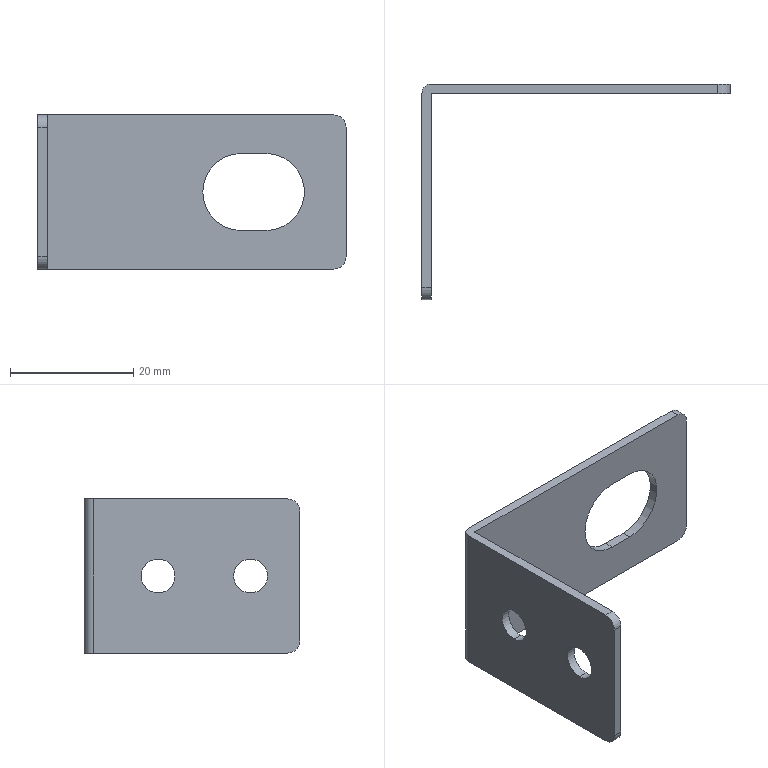Component | SolidWorks | SensorFixingBlock-1 | 1 solid | 22 faces | box 50 x 35 x 25 mm | volume 2784 mm3 | cylinder 12 | plane 10 | commonest cylinder face diameters 5.5 x4 4 x4 12.5 x3 3 x1 | material Plain Carbon Steel
build123d program:
from build123d import *

# Parameters (mm, degrees)
EXTRUDE_THIN1_DEPTH = 12.5
FILLET1_R           = 1.5
FILLET2_R           = 2
CUT_EXTRUDE1_DEPTH  = 63.3
SKETCH3_R           = 2.75
CUT_EXTRUDE2_DEPTH  = 63.3


with BuildPart() as part:
    # Sketch1 → Extrude-Thin1 (new, symmetric)
    with BuildSketch(Plane.XY):
        Polygon((0, 50), (0, 0), (35, 0), (35, 1.5), (1.5, 1.5), (1.5, 50), align=None)
    extrude(amount=EXTRUDE_THIN1_DEPTH, both=True)

    # Fillet1
    fillet1_edges = [part.edges().sort_by_distance(p)[0] for p in [
        (0, 0, 0),
    ]]
    fillet(fillet1_edges, radius=FILLET1_R)

    # Fillet2
    fillet2_edges = [part.edges().sort_by_distance(p)[0] for p in [
        (0.75, 50, 12.5),
        (0.75, 50, -12.5),
        (35, 0.75, -12.5),
        (35, 0.75, 12.5),
    ]]
    fillet(fillet2_edges, radius=FILLET2_R)

    # Sketch2 → Cut-Extrude1 (cut, through all)
    with BuildSketch(Plane.ZY):
        with BuildLine():
            Line((-6.25, 33), (-6.25, 37))
            ThreePointArc((-6.25, 37), (0, 43.25), (6.25, 37))
            Line((6.25, 37), (6.25, 33))
            ThreePointArc((6.25, 33), (0, 26.75), (-6.25, 33))
        make_face()
    extrude(amount=-CUT_EXTRUDE1_DEPTH, mode=Mode.SUBTRACT)

    # Sketch3 → Cut-Extrude2 (cut, through all)
    with BuildSketch(Plane.XZ):
        with Locations(Location((12, 0, 0), (0, 0, 270))):
            Circle(SKETCH3_R)
        with Locations(Location((27, 0, 0), (0, 0, 270))):
            Circle(SKETCH3_R)
    extrude(amount=-CUT_EXTRUDE2_DEPTH, mode=Mode.SUBTRACT)


solid = part.part

# Placed as in the assembly
solid = solid.moved(Location((-129.666, 17.264, 37), (0, 0, -90)))
STEP:
#1=COLOUR_RGB('',0.7922,0.8196,0.9333);
#2=FILL_AREA_STYLE_COLOUR('',#1);
#3=FILL_AREA_STYLE('',(#2));
#4=SURFACE_STYLE_FILL_AREA(#3);
#5=SURFACE_SIDE_STYLE('',(#4));
#6=SURFACE_STYLE_USAGE(.BOTH.,#5);
#7=PRESENTATION_STYLE_ASSIGNMENT((#6));
#8=CARTESIAN_POINT('',(-5.046,-0.3833,1.348));
#9=VERTEX_POINT('',#8);
#10=CARTESIAN_POINT('',(-5.046,-0.3833,1.565));
#11=VERTEX_POINT('',#10);
#12=CARTESIAN_POINT('',(-5.046,-0.3833,1.457));
#13=DIRECTION('',(1.,-0.,0.));
#14=DIRECTION('',(0.,0.,1.));
#15=AXIS2_PLACEMENT_3D('',#12,#13,#14);
#16=CIRCLE('',#15,0.1083);
#17=EDGE_CURVE('',#9,#11,#16,.T.);
#18=ORIENTED_EDGE('',*,*,#17,.T.);
#19=CARTESIAN_POINT('',(-5.105,-0.3833,1.565));
#20=VERTEX_POINT('',#19);
#21=CARTESIAN_POINT('',(-3.136,-0.3833,1.565));
#22=DIRECTION('',(-1.,0.,0.));
#23=VECTOR('',#22,39.37);
#24=LINE('',#21,#23);
#25=EDGE_CURVE('',#11,#20,#24,.T.);
#26=ORIENTED_EDGE('',*,*,#25,.T.);
#27=CARTESIAN_POINT('',(-5.105,-0.3833,1.348));
#28=VERTEX_POINT('',#27);
#29=CARTESIAN_POINT('',(-5.105,-0.3833,1.457));
#30=DIRECTION('',(-1.,0.,0.));
#31=DIRECTION('',(0.,0.,-1.));
#32=AXIS2_PLACEMENT_3D('',#29,#30,#31);
#33=CIRCLE('',#32,0.1083);
#34=EDGE_CURVE('',#20,#28,#33,.T.);
#35=ORIENTED_EDGE('',*,*,#34,.T.);
#36=CARTESIAN_POINT('',(-3.136,-0.3833,1.348));
#37=DIRECTION('',(-1.,0.,0.));
#38=VECTOR('',#37,39.37);
#39=LINE('',#36,#38);
#40=EDGE_CURVE('',#9,#28,#39,.T.);
#41=ORIENTED_EDGE('',*,*,#40,.F.);
#42=EDGE_LOOP('',(#18,#26,#35,#41));
#43=FACE_OUTER_BOUND('',#42,.T.);
#44=CARTESIAN_POINT('',(-3.136,-0.3833,1.457));
#45=DIRECTION('',(-1.,0.,0.));
#46=DIRECTION('',(0.,0.,-1.));
#47=AXIS2_PLACEMENT_3D('',#44,#45,#46);
#48=CYLINDRICAL_SURFACE('',#47,0.1083);
#49=ADVANCED_FACE('',(#43),#48,.F.);
#50=CARTESIAN_POINT('',(-5.046,0.2072,1.348));
#51=VERTEX_POINT('',#50);
#52=CARTESIAN_POINT('',(-5.046,0.2072,1.565));
#53=VERTEX_POINT('',#52);
#54=CARTESIAN_POINT('',(-5.046,0.2072,1.457));
#55=DIRECTION('',(1.,-0.,0.));
#56=DIRECTION('',(0.,0.,1.));
#57=AXIS2_PLACEMENT_3D('',#54,#55,#56);
#58=CIRCLE('',#57,0.1083);
#59=EDGE_CURVE('',#51,#53,#58,.T.);
#60=ORIENTED_EDGE('',*,*,#59,.T.);
#61=CARTESIAN_POINT('',(-5.105,0.2072,1.565));
#62=VERTEX_POINT('',#61);
#63=CARTESIAN_POINT('',(-3.136,0.2072,1.565));
#64=DIRECTION('',(-1.,0.,0.));
#65=VECTOR('',#64,39.37);
#66=LINE('',#63,#65);
#67=EDGE_CURVE('',#53,#62,#66,.T.);
#68=ORIENTED_EDGE('',*,*,#67,.T.);
#69=CARTESIAN_POINT('',(-5.105,0.2072,1.348));
#70=VERTEX_POINT('',#69);
#71=CARTESIAN_POINT('',(-5.105,0.2072,1.457));
#72=DIRECTION('',(-1.,0.,0.));
#73=DIRECTION('',(0.,0.,-1.));
#74=AXIS2_PLACEMENT_3D('',#71,#72,#73);
#75=CIRCLE('',#74,0.1083);
#76=EDGE_CURVE('',#62,#70,#75,.T.);
#77=ORIENTED_EDGE('',*,*,#76,.T.);
#78=CARTESIAN_POINT('',(-3.136,0.2072,1.348));
#79=DIRECTION('',(-1.,0.,0.));
#80=VECTOR('',#79,39.37);
#81=LINE('',#78,#80);
#82=EDGE_CURVE('',#51,#70,#81,.T.);
#83=ORIENTED_EDGE('',*,*,#82,.F.);
#84=EDGE_LOOP('',(#60,#68,#77,#83));
#85=FACE_OUTER_BOUND('',#84,.T.);
#86=CARTESIAN_POINT('',(-3.136,0.2072,1.457));
#87=DIRECTION('',(-1.,0.,0.));
#88=DIRECTION('',(0.,0.,-1.));
#89=AXIS2_PLACEMENT_3D('',#86,#87,#88);
#90=CYLINDRICAL_SURFACE('',#89,0.1083);
#91=ADVANCED_FACE('',(#85),#90,.F.);
#92=CARTESIAN_POINT('',(-3.806,0.6206,1.703));
#93=VERTEX_POINT('',#92);
#94=CARTESIAN_POINT('',(-4.052,0.6206,1.457));
#95=VERTEX_POINT('',#94);
#96=CARTESIAN_POINT('',(-3.806,0.6206,1.457));
#97=DIRECTION('',(-0.,-1.,0.));
#98=DIRECTION('',(1.,0.,0.));
#99=AXIS2_PLACEMENT_3D('',#96,#97,#98);
#100=CIRCLE('',#99,0.2461);
#101=EDGE_CURVE('',#93,#95,#100,.T.);
#102=ORIENTED_EDGE('',*,*,#101,.T.);
#103=CARTESIAN_POINT('',(-4.052,0.6797,1.457));
#104=VERTEX_POINT('',#103);
#105=CARTESIAN_POINT('',(-4.052,-0.6983,1.457));
#106=DIRECTION('',(0.,1.,0.));
#107=VECTOR('',#106,39.37);
#108=LINE('',#105,#107);
#109=EDGE_CURVE('',#95,#104,#108,.T.);
#110=ORIENTED_EDGE('',*,*,#109,.T.);
#111=CARTESIAN_POINT('',(-3.806,0.6797,1.703));
#112=VERTEX_POINT('',#111);
#113=CARTESIAN_POINT('',(-3.806,0.6797,1.457));
#114=DIRECTION('',(0.,1.,0.));
#115=DIRECTION('',(-1.,0.,0.));
#116=AXIS2_PLACEMENT_3D('',#113,#114,#115);
#117=CIRCLE('',#116,0.2461);
#118=EDGE_CURVE('',#104,#112,#117,.T.);
#119=ORIENTED_EDGE('',*,*,#118,.T.);
#120=CARTESIAN_POINT('',(-3.806,-0.6983,1.703));
#121=DIRECTION('',(0.,1.,0.));
#122=VECTOR('',#121,39.37);
#123=LINE('',#120,#122);
#124=EDGE_CURVE('',#93,#112,#123,.T.);
#125=ORIENTED_EDGE('',*,*,#124,.F.);
#126=EDGE_LOOP('',(#102,#110,#119,#125));
#127=FACE_OUTER_BOUND('',#126,.T.);
#128=CARTESIAN_POINT('',(-3.806,-0.6983,1.457));
#129=DIRECTION('',(0.,1.,0.));
#130=DIRECTION('',(-1.,0.,0.));
#131=AXIS2_PLACEMENT_3D('',#128,#129,#130);
#132=CYLINDRICAL_SURFACE('',#131,0.2461);
#133=ADVANCED_FACE('',(#127),#132,.F.);
#134=CARTESIAN_POINT('',(-5.105,-0.3833,1.457));
#135=DIRECTION('',(-1.,0.,0.));
#136=DIRECTION('',(0.,0.,-1.));
#137=AXIS2_PLACEMENT_3D('',#134,#135,#136);
#138=CIRCLE('',#137,0.1083);
#139=EDGE_CURVE('',#28,#20,#138,.T.);
#140=ORIENTED_EDGE('',*,*,#139,.F.);
#141=ORIENTED_EDGE('',*,*,#34,.F.);
#142=EDGE_LOOP('',(#140,#141));
#143=FACE_BOUND('',#142,.T.);
#144=CARTESIAN_POINT('',(-5.105,0.2072,1.457));
#145=DIRECTION('',(-1.,0.,0.));
#146=DIRECTION('',(0.,0.,-1.));
#147=AXIS2_PLACEMENT_3D('',#144,#145,#146);
#148=CIRCLE('',#147,0.1083);
#149=EDGE_CURVE('',#70,#62,#148,.T.);
#150=ORIENTED_EDGE('',*,*,#149,.F.);
#151=ORIENTED_EDGE('',*,*,#76,.F.);
#152=EDGE_LOOP('',(#150,#151));
#153=FACE_BOUND('',#152,.T.);
#154=CARTESIAN_POINT('',(-5.105,0.6206,0.9646));
#155=VERTEX_POINT('',#154);
#156=CARTESIAN_POINT('',(-5.105,-0.6195,0.9646));
#157=VERTEX_POINT('',#156);
#158=CARTESIAN_POINT('',(-5.105,0.6797,0.9646));
#159=DIRECTION('',(-0.,-1.,0.));
#160=VECTOR('',#159,39.37);
#161=LINE('',#158,#160);
#162=EDGE_CURVE('',#155,#157,#161,.T.);
#163=ORIENTED_EDGE('',*,*,#162,.T.);
#164=CARTESIAN_POINT('',(-5.105,-0.6983,1.043));
#165=VERTEX_POINT('',#164);
#166=CARTESIAN_POINT('',(-5.105,-0.6195,1.043));
#167=DIRECTION('',(-1.,0.,0.));
#168=DIRECTION('',(0.,0.,1.));
#169=AXIS2_PLACEMENT_3D('',#166,#167,#168);
#170=CIRCLE('',#169,0.07874);
#171=EDGE_CURVE('',#157,#165,#170,.T.);
#172=ORIENTED_EDGE('',*,*,#171,.T.);
#173=CARTESIAN_POINT('',(-5.105,-0.6983,1.87));
#174=VERTEX_POINT('',#173);
#175=CARTESIAN_POINT('',(-5.105,-0.6983,1.949));
#176=DIRECTION('',(0.,0.,-1.));
#177=VECTOR('',#176,39.37);
#178=LINE('',#175,#177);
#179=EDGE_CURVE('',#174,#165,#178,.T.);
#180=ORIENTED_EDGE('',*,*,#179,.F.);
#181=CARTESIAN_POINT('',(-5.105,-0.6195,1.949));
#182=VERTEX_POINT('',#181);
#183=CARTESIAN_POINT('',(-5.105,-0.6195,1.87));
#184=DIRECTION('',(-1.,0.,0.));
#185=DIRECTION('',(0.,0.,1.));
#186=AXIS2_PLACEMENT_3D('',#183,#184,#185);
#187=CIRCLE('',#186,0.07874);
#188=EDGE_CURVE('',#174,#182,#187,.T.);
#189=ORIENTED_EDGE('',*,*,#188,.T.);
#190=CARTESIAN_POINT('',(-5.105,0.6206,1.949));
#191=VERTEX_POINT('',#190);
#192=CARTESIAN_POINT('',(-5.105,0.6797,1.949));
#193=DIRECTION('',(-0.,-1.,0.));
#194=VECTOR('',#193,39.37);
#195=LINE('',#192,#194);
#196=EDGE_CURVE('',#191,#182,#195,.T.);
#197=ORIENTED_EDGE('',*,*,#196,.F.);
#198=CARTESIAN_POINT('',(-5.105,0.6206,1.949));
#199=DIRECTION('',(0.,0.,-1.));
#200=VECTOR('',#199,39.37);
#201=LINE('',#198,#200);
#202=EDGE_CURVE('',#191,#155,#201,.T.);
#203=ORIENTED_EDGE('',*,*,#202,.T.);
#204=EDGE_LOOP('',(#163,#172,#180,#189,#197,#203));
#205=FACE_OUTER_BOUND('',#204,.T.);
#206=CARTESIAN_POINT('',(-5.105,0.6797,1.949));
#207=DIRECTION('',(1.,-0.,0.));
#208=DIRECTION('',(0.,0.,1.));
#209=AXIS2_PLACEMENT_3D('',#206,#207,#208);
#210=PLANE('',#209);
#211=ADVANCED_FACE('',(#143,#153,#205),#210,.F.);
#212=ORIENTED_EDGE('',*,*,#179,.T.);
#213=CARTESIAN_POINT('',(-5.046,-0.6983,1.043));
#214=VERTEX_POINT('',#213);
#215=CARTESIAN_POINT('',(-5.046,-0.6983,1.043));
#216=DIRECTION('',(1.,-0.,0.));
#217=VECTOR('',#216,39.37);
#218=LINE('',#215,#217);
#219=EDGE_CURVE('',#165,#214,#218,.T.);
#220=ORIENTED_EDGE('',*,*,#219,.T.);
#221=CARTESIAN_POINT('',(-5.046,-0.6983,1.87));
#222=VERTEX_POINT('',#221);
#223=CARTESIAN_POINT('',(-5.046,-0.6983,1.949));
#224=DIRECTION('',(0.,0.,-1.));
#225=VECTOR('',#224,39.37);
#226=LINE('',#223,#225);
#227=EDGE_CURVE('',#222,#214,#226,.T.);
#228=ORIENTED_EDGE('',*,*,#227,.F.);
#229=CARTESIAN_POINT('',(-5.105,-0.6983,1.87));
#230=DIRECTION('',(-1.,0.,0.));
#231=VECTOR('',#230,39.37);
#232=LINE('',#229,#231);
#233=EDGE_CURVE('',#222,#174,#232,.T.);
#234=ORIENTED_EDGE('',*,*,#233,.T.);
#235=EDGE_LOOP('',(#212,#220,#228,#234));
#236=FACE_OUTER_BOUND('',#235,.T.);
#237=CARTESIAN_POINT('',(-5.046,-0.6983,1.949));
#238=DIRECTION('',(-0.,-1.,0.));
#239=DIRECTION('',(0.,0.,-1.));
#240=AXIS2_PLACEMENT_3D('',#237,#238,#239);
#241=PLANE('',#240);
#242=ADVANCED_FACE('',(#236),#241,.T.);
#243=ORIENTED_EDGE('',*,*,#17,.F.);
#244=CARTESIAN_POINT('',(-5.046,-0.3833,1.457));
#245=DIRECTION('',(1.,-0.,0.));
#246=DIRECTION('',(0.,0.,1.));
#247=AXIS2_PLACEMENT_3D('',#244,#245,#246);
#248=CIRCLE('',#247,0.1083);
#249=EDGE_CURVE('',#11,#9,#248,.T.);
#250=ORIENTED_EDGE('',*,*,#249,.F.);
#251=EDGE_LOOP('',(#243,#250));
#252=FACE_BOUND('',#251,.T.);
#253=ORIENTED_EDGE('',*,*,#59,.F.);
#254=CARTESIAN_POINT('',(-5.046,0.2072,1.457));
#255=DIRECTION('',(1.,-0.,0.));
#256=DIRECTION('',(0.,0.,1.));
#257=AXIS2_PLACEMENT_3D('',#254,#255,#256);
#258=CIRCLE('',#257,0.1083);
#259=EDGE_CURVE('',#53,#51,#258,.T.);
#260=ORIENTED_EDGE('',*,*,#259,.F.);
#261=EDGE_LOOP('',(#253,#260));
#262=FACE_BOUND('',#261,.T.);
#263=ORIENTED_EDGE('',*,*,#227,.T.);
#264=CARTESIAN_POINT('',(-5.046,-0.6195,0.9646));
#265=VERTEX_POINT('',#264);
#266=CARTESIAN_POINT('',(-5.046,-0.6195,1.043));
#267=DIRECTION('',(1.,-0.,0.));
#268=DIRECTION('',(0.,0.,1.));
#269=AXIS2_PLACEMENT_3D('',#266,#267,#268);
#270=CIRCLE('',#269,0.07874);
#271=EDGE_CURVE('',#214,#265,#270,.T.);
#272=ORIENTED_EDGE('',*,*,#271,.T.);
#273=CARTESIAN_POINT('',(-5.046,0.6206,0.9646));
#274=VERTEX_POINT('',#273);
#275=CARTESIAN_POINT('',(-5.046,0.6797,0.9646));
#276=DIRECTION('',(-0.,-1.,0.));
#277=VECTOR('',#276,39.37);
#278=LINE('',#275,#277);
#279=EDGE_CURVE('',#274,#265,#278,.T.);
#280=ORIENTED_EDGE('',*,*,#279,.F.);
#281=CARTESIAN_POINT('',(-5.046,0.6206,1.949));
#282=VERTEX_POINT('',#281);
#283=CARTESIAN_POINT('',(-5.046,0.6206,1.949));
#284=DIRECTION('',(0.,0.,-1.));
#285=VECTOR('',#284,39.37);
#286=LINE('',#283,#285);
#287=EDGE_CURVE('',#282,#274,#286,.T.);
#288=ORIENTED_EDGE('',*,*,#287,.F.);
#289=CARTESIAN_POINT('',(-5.046,-0.6195,1.949));
#290=VERTEX_POINT('',#289);
#291=CARTESIAN_POINT('',(-5.046,0.6797,1.949));
#292=DIRECTION('',(-0.,-1.,0.));
#293=VECTOR('',#292,39.37);
#294=LINE('',#291,#293);
#295=EDGE_CURVE('',#282,#290,#294,.T.);
#296=ORIENTED_EDGE('',*,*,#295,.T.);
#297=CARTESIAN_POINT('',(-5.046,-0.6195,1.87));
#298=DIRECTION('',(1.,-0.,0.));
#299=DIRECTION('',(0.,0.,1.));
#300=AXIS2_PLACEMENT_3D('',#297,#298,#299);
#301=CIRCLE('',#300,0.07874);
#302=EDGE_CURVE('',#290,#222,#301,.T.);
#303=ORIENTED_EDGE('',*,*,#302,.T.);
#304=EDGE_LOOP('',(#263,#272,#280,#288,#296,#303));
#305=FACE_OUTER_BOUND('',#304,.T.);
#306=CARTESIAN_POINT('',(-5.046,0.6797,1.949));
#307=DIRECTION('',(1.,-0.,0.));
#308=DIRECTION('',(0.,0.,1.));
#309=AXIS2_PLACEMENT_3D('',#306,#307,#308);
#310=PLANE('',#309);
#311=ADVANCED_FACE('',(#252,#262,#305),#310,.T.);
#312=ORIENTED_EDGE('',*,*,#101,.F.);
#313=CARTESIAN_POINT('',(-3.648,0.6206,1.703));
#314=VERTEX_POINT('',#313);
#315=CARTESIAN_POINT('',(-3.136,0.6206,1.703));
#316=DIRECTION('',(-1.,0.,0.));
#317=VECTOR('',#316,39.37);
#318=LINE('',#315,#317);
#319=EDGE_CURVE('',#314,#93,#318,.T.);
#320=ORIENTED_EDGE('',*,*,#319,.F.);
#321=CARTESIAN_POINT('',(-3.648,0.6206,1.211));
#322=VERTEX_POINT('',#321);
#323=CARTESIAN_POINT('',(-3.648,0.6206,1.457));
#324=DIRECTION('',(-0.,-1.,0.));
#325=DIRECTION('',(1.,0.,0.));
#326=AXIS2_PLACEMENT_3D('',#323,#324,#325);
#327=CIRCLE('',#326,0.2461);
#328=EDGE_CURVE('',#322,#314,#327,.T.);
#329=ORIENTED_EDGE('',*,*,#328,.F.);
#330=CARTESIAN_POINT('',(-3.806,0.6206,1.211));
#331=VERTEX_POINT('',#330);
#332=CARTESIAN_POINT('',(-3.136,0.6206,1.211));
#333=DIRECTION('',(1.,-0.,-0.));
#334=VECTOR('',#333,39.37);
#335=LINE('',#332,#334);
#336=EDGE_CURVE('',#331,#322,#335,.T.);
#337=ORIENTED_EDGE('',*,*,#336,.F.);
#338=CARTESIAN_POINT('',(-3.806,0.6206,1.457));
#339=DIRECTION('',(-0.,-1.,0.));
#340=DIRECTION('',(1.,0.,0.));
#341=AXIS2_PLACEMENT_3D('',#338,#339,#340);
#342=CIRCLE('',#341,0.2461);
#343=EDGE_CURVE('',#95,#331,#342,.T.);
#344=ORIENTED_EDGE('',*,*,#343,.F.);
#345=EDGE_LOOP('',(#312,#320,#329,#337,#344));
#346=FACE_BOUND('',#345,.T.);
#347=CARTESIAN_POINT('',(-3.215,0.6206,0.9646));
#348=VERTEX_POINT('',#347);
#349=CARTESIAN_POINT('',(-3.136,0.6206,0.9646));
#350=DIRECTION('',(-1.,0.,0.));
#351=VECTOR('',#350,39.37);
#352=LINE('',#349,#351);
#353=EDGE_CURVE('',#348,#274,#352,.T.);
#354=ORIENTED_EDGE('',*,*,#353,.F.);
#355=CARTESIAN_POINT('',(-3.136,0.6206,1.043));
#356=VERTEX_POINT('',#355);
#357=CARTESIAN_POINT('',(-3.215,0.6206,1.043));
#358=DIRECTION('',(-0.,-1.,0.));
#359=DIRECTION('',(1.,0.,0.));
#360=AXIS2_PLACEMENT_3D('',#357,#358,#359);
#361=CIRCLE('',#360,0.07874);
#362=EDGE_CURVE('',#348,#356,#361,.T.);
#363=ORIENTED_EDGE('',*,*,#362,.T.);
#364=CARTESIAN_POINT('',(-3.136,0.6206,1.87));
#365=VERTEX_POINT('',#364);
#366=CARTESIAN_POINT('',(-3.136,0.6206,1.949));
#367=DIRECTION('',(0.,0.,-1.));
#368=VECTOR('',#367,39.37);
#369=LINE('',#366,#368);
#370=EDGE_CURVE('',#365,#356,#369,.T.);
#371=ORIENTED_EDGE('',*,*,#370,.F.);
#372=CARTESIAN_POINT('',(-3.215,0.6206,1.949));
#373=VERTEX_POINT('',#372);
#374=CARTESIAN_POINT('',(-3.215,0.6206,1.87));
#375=DIRECTION('',(-0.,-1.,0.));
#376=DIRECTION('',(1.,0.,0.));
#377=AXIS2_PLACEMENT_3D('',#374,#375,#376);
#378=CIRCLE('',#377,0.07874);
#379=EDGE_CURVE('',#365,#373,#378,.T.);
#380=ORIENTED_EDGE('',*,*,#379,.T.);
#381=CARTESIAN_POINT('',(-3.136,0.6206,1.949));
#382=DIRECTION('',(-1.,0.,0.));
#383=VECTOR('',#382,39.37);
#384=LINE('',#381,#383);
#385=EDGE_CURVE('',#373,#282,#384,.T.);
#386=ORIENTED_EDGE('',*,*,#385,.T.);
#387=ORIENTED_EDGE('',*,*,#287,.T.);
#388=EDGE_LOOP('',(#354,#363,#371,#380,#386,#387));
#389=FACE_OUTER_BOUND('',#388,.T.);
#390=CARTESIAN_POINT('',(-3.136,0.6206,1.949));
#391=DIRECTION('',(-0.,-1.,0.));
#392=DIRECTION('',(1.,-0.,0.));
#393=AXIS2_PLACEMENT_3D('',#390,#391,#392);
#394=PLANE('',#393);
#395=ADVANCED_FACE('',(#346,#389),#394,.T.);
#396=ORIENTED_EDGE('',*,*,#370,.T.);
#397=CARTESIAN_POINT('',(-3.136,0.6797,1.043));
#398=VERTEX_POINT('',#397);
#399=CARTESIAN_POINT('',(-3.136,0.6797,1.043));
#400=DIRECTION('',(0.,1.,0.));
#401=VECTOR('',#400,39.37);
#402=LINE('',#399,#401);
#403=EDGE_CURVE('',#356,#398,#402,.T.);
#404=ORIENTED_EDGE('',*,*,#403,.T.);
#405=CARTESIAN_POINT('',(-3.136,0.6797,1.87));
#406=VERTEX_POINT('',#405);
#407=CARTESIAN_POINT('',(-3.136,0.6797,1.949));
#408=DIRECTION('',(0.,0.,-1.));
#409=VECTOR('',#408,39.37);
#410=LINE('',#407,#409);
#411=EDGE_CURVE('',#406,#398,#410,.T.);
#412=ORIENTED_EDGE('',*,*,#411,.F.);
#413=CARTESIAN_POINT('',(-3.136,0.6206,1.87));
#414=DIRECTION('',(-0.,-1.,0.));
#415=VECTOR('',#414,39.37);
#416=LINE('',#413,#415);
#417=EDGE_CURVE('',#406,#365,#416,.T.);
#418=ORIENTED_EDGE('',*,*,#417,.T.);
#419=EDGE_LOOP('',(#396,#404,#412,#418));
#420=FACE_OUTER_BOUND('',#419,.T.);
#421=CARTESIAN_POINT('',(-3.136,0.6797,1.949));
#422=DIRECTION('',(1.,-0.,0.));
#423=DIRECTION('',(0.,0.,1.));
#424=AXIS2_PLACEMENT_3D('',#421,#422,#423);
#425=PLANE('',#424);
#426=ADVANCED_FACE('',(#420),#425,.T.);
#427=CARTESIAN_POINT('',(-3.648,0.6797,1.703));
#428=VERTEX_POINT('',#427);
#429=CARTESIAN_POINT('',(-3.806,0.6797,1.703));
#430=DIRECTION('',(1.,-0.,-0.));
#431=VECTOR('',#430,39.37);
#432=LINE('',#429,#431);
#433=EDGE_CURVE('',#112,#428,#432,.T.);
#434=ORIENTED_EDGE('',*,*,#433,.F.);
#435=ORIENTED_EDGE('',*,*,#118,.F.);
#436=CARTESIAN_POINT('',(-3.806,0.6797,1.211));
#437=VERTEX_POINT('',#436);
#438=CARTESIAN_POINT('',(-3.806,0.6797,1.457));
#439=DIRECTION('',(0.,1.,0.));
#440=DIRECTION('',(-1.,0.,0.));
#441=AXIS2_PLACEMENT_3D('',#438,#439,#440);
#442=CIRCLE('',#441,0.2461);
#443=EDGE_CURVE('',#437,#104,#442,.T.);
#444=ORIENTED_EDGE('',*,*,#443,.F.);
#445=CARTESIAN_POINT('',(-3.648,0.6797,1.211));
#446=VERTEX_POINT('',#445);
#447=CARTESIAN_POINT('',(-3.806,0.6797,1.211));
#448=DIRECTION('',(-1.,0.,0.));
#449=VECTOR('',#448,39.37);
#450=LINE('',#447,#449);
#451=EDGE_CURVE('',#446,#437,#450,.T.);
#452=ORIENTED_EDGE('',*,*,#451,.F.);
#453=CARTESIAN_POINT('',(-3.648,0.6797,1.457));
#454=DIRECTION('',(0.,1.,0.));
#455=DIRECTION('',(-1.,0.,0.));
#456=AXIS2_PLACEMENT_3D('',#453,#454,#455);
#457=CIRCLE('',#456,0.2461);
#458=EDGE_CURVE('',#428,#446,#457,.T.);
#459=ORIENTED_EDGE('',*,*,#458,.F.);
#460=EDGE_LOOP('',(#434,#435,#444,#452,#459));
#461=FACE_BOUND('',#460,.T.);
#462=ORIENTED_EDGE('',*,*,#411,.T.);
#463=CARTESIAN_POINT('',(-3.215,0.6797,0.9646));
#464=VERTEX_POINT('',#463);
#465=CARTESIAN_POINT('',(-3.215,0.6797,1.043));
#466=DIRECTION('',(0.,1.,0.));
#467=DIRECTION('',(1.,0.,0.));
#468=AXIS2_PLACEMENT_3D('',#465,#466,#467);
#469=CIRCLE('',#468,0.07874);
#470=EDGE_CURVE('',#398,#464,#469,.T.);
#471=ORIENTED_EDGE('',*,*,#470,.T.);
#472=CARTESIAN_POINT('',(-5.046,0.6797,0.9646));
#473=VERTEX_POINT('',#472);
#474=CARTESIAN_POINT('',(-3.136,0.6797,0.9646));
#475=DIRECTION('',(-1.,0.,0.));
#476=VECTOR('',#475,39.37);
#477=LINE('',#474,#476);
#478=EDGE_CURVE('',#464,#473,#477,.T.);
#479=ORIENTED_EDGE('',*,*,#478,.T.);
#480=CARTESIAN_POINT('',(-5.046,0.6797,1.949));
#481=VERTEX_POINT('',#480);
#482=CARTESIAN_POINT('',(-5.046,0.6797,1.949));
#483=DIRECTION('',(0.,0.,1.));
#484=VECTOR('',#483,39.37);
#485=LINE('',#482,#484);
#486=EDGE_CURVE('',#473,#481,#485,.T.);
#487=ORIENTED_EDGE('',*,*,#486,.T.);
#488=CARTESIAN_POINT('',(-3.215,0.6797,1.949));
#489=VERTEX_POINT('',#488);
#490=CARTESIAN_POINT('',(-3.136,0.6797,1.949));
#491=DIRECTION('',(-1.,0.,0.));
#492=VECTOR('',#491,39.37);
#493=LINE('',#490,#492);
#494=EDGE_CURVE('',#489,#481,#493,.T.);
#495=ORIENTED_EDGE('',*,*,#494,.F.);
#496=CARTESIAN_POINT('',(-3.215,0.6797,1.87));
#497=DIRECTION('',(0.,1.,0.));
#498=DIRECTION('',(1.,0.,0.));
#499=AXIS2_PLACEMENT_3D('',#496,#497,#498);
#500=CIRCLE('',#499,0.07874);
#501=EDGE_CURVE('',#489,#406,#500,.T.);
#502=ORIENTED_EDGE('',*,*,#501,.T.);
#503=EDGE_LOOP('',(#462,#471,#479,#487,#495,#502));
#504=FACE_OUTER_BOUND('',#503,.T.);
#505=CARTESIAN_POINT('',(-3.136,0.6797,1.949));
#506=DIRECTION('',(-0.,-1.,0.));
#507=DIRECTION('',(1.,-0.,0.));
#508=AXIS2_PLACEMENT_3D('',#505,#506,#507);
#509=PLANE('',#508);
#510=ADVANCED_FACE('',(#461,#504),#509,.F.);
#511=ORIENTED_EDGE('',*,*,#385,.F.);
#512=CARTESIAN_POINT('',(-3.215,0.6797,1.949));
#513=DIRECTION('',(0.,1.,0.));
#514=VECTOR('',#513,39.37);
#515=LINE('',#512,#514);
#516=EDGE_CURVE('',#373,#489,#515,.T.);
#517=ORIENTED_EDGE('',*,*,#516,.T.);
#518=ORIENTED_EDGE('',*,*,#494,.T.);
#519=CARTESIAN_POINT('',(-5.046,0.6206,1.949));
#520=DIRECTION('',(0.,0.,1.));
#521=DIRECTION('',(0.,1.,0.));
#522=AXIS2_PLACEMENT_3D('',#519,#520,#521);
#523=CIRCLE('',#522,0.05906);
#524=EDGE_CURVE('',#481,#191,#523,.T.);
#525=ORIENTED_EDGE('',*,*,#524,.T.);
#526=ORIENTED_EDGE('',*,*,#196,.T.);
#527=CARTESIAN_POINT('',(-5.046,-0.6195,1.949));
#528=DIRECTION('',(1.,-0.,0.));
#529=VECTOR('',#528,39.37);
#530=LINE('',#527,#529);
#531=EDGE_CURVE('',#182,#290,#530,.T.);
#532=ORIENTED_EDGE('',*,*,#531,.T.);
#533=ORIENTED_EDGE('',*,*,#295,.F.);
#534=EDGE_LOOP('',(#511,#517,#518,#525,#526,#532,#533));
#535=FACE_OUTER_BOUND('',#534,.T.);
#536=CARTESIAN_POINT('',(-5.105,0.6797,1.949));
#537=DIRECTION('',(0.,0.,-1.));
#538=DIRECTION('',(0.,1.,0.));
#539=AXIS2_PLACEMENT_3D('',#536,#537,#538);
#540=PLANE('',#539);
#541=ADVANCED_FACE('',(#535),#540,.F.);
#542=ORIENTED_EDGE('',*,*,#478,.F.);
#543=CARTESIAN_POINT('',(-3.215,0.6797,0.9646));
#544=DIRECTION('',(-0.,-1.,0.));
#545=VECTOR('',#544,39.37);
#546=LINE('',#543,#545);
#547=EDGE_CURVE('',#464,#348,#546,.T.);
#548=ORIENTED_EDGE('',*,*,#547,.T.);
#549=ORIENTED_EDGE('',*,*,#353,.T.);
#550=ORIENTED_EDGE('',*,*,#279,.T.);
#551=CARTESIAN_POINT('',(-5.105,-0.6195,0.9646));
#552=DIRECTION('',(-1.,0.,0.));
#553=VECTOR('',#552,39.37);
#554=LINE('',#551,#553);
#555=EDGE_CURVE('',#265,#157,#554,.T.);
#556=ORIENTED_EDGE('',*,*,#555,.T.);
#557=ORIENTED_EDGE('',*,*,#162,.F.);
#558=CARTESIAN_POINT('',(-5.046,0.6206,0.9646));
#559=DIRECTION('',(0.,0.,-1.));
#560=DIRECTION('',(0.,1.,0.));
#561=AXIS2_PLACEMENT_3D('',#558,#559,#560);
#562=CIRCLE('',#561,0.05906);
#563=EDGE_CURVE('',#155,#473,#562,.T.);
#564=ORIENTED_EDGE('',*,*,#563,.T.);
#565=EDGE_LOOP('',(#542,#548,#549,#550,#556,#557,#564));
#566=FACE_OUTER_BOUND('',#565,.T.);
#567=CARTESIAN_POINT('',(-5.105,0.6797,0.9646));
#568=DIRECTION('',(0.,0.,-1.));
#569=DIRECTION('',(0.,1.,0.));
#570=AXIS2_PLACEMENT_3D('',#567,#568,#569);
#571=PLANE('',#570);
#572=ADVANCED_FACE('',(#566),#571,.T.);
#573=ORIENTED_EDGE('',*,*,#524,.F.);
#574=ORIENTED_EDGE('',*,*,#486,.F.);
#575=ORIENTED_EDGE('',*,*,#563,.F.);
#576=ORIENTED_EDGE('',*,*,#202,.F.);
#577=EDGE_LOOP('',(#573,#574,#575,#576));
#578=FACE_OUTER_BOUND('',#577,.T.);
#579=CARTESIAN_POINT('',(-5.046,0.6206,1.949));
#580=DIRECTION('',(0.,0.,-1.));
#581=DIRECTION('',(0.,1.,0.));
#582=AXIS2_PLACEMENT_3D('',#579,#580,#581);
#583=CYLINDRICAL_SURFACE('',#582,0.05906);
#584=ADVANCED_FACE('',(#578),#583,.T.);
#585=ORIENTED_EDGE('',*,*,#470,.F.);
#586=ORIENTED_EDGE('',*,*,#403,.F.);
#587=ORIENTED_EDGE('',*,*,#362,.F.);
#588=ORIENTED_EDGE('',*,*,#547,.F.);
#589=EDGE_LOOP('',(#585,#586,#587,#588));
#590=FACE_OUTER_BOUND('',#589,.T.);
#591=CARTESIAN_POINT('',(-3.215,0.6797,1.043));
#592=DIRECTION('',(-0.,-1.,0.));
#593=DIRECTION('',(0.,0.,-1.));
#594=AXIS2_PLACEMENT_3D('',#591,#592,#593);
#595=CYLINDRICAL_SURFACE('',#594,0.07874);
#596=ADVANCED_FACE('',(#590),#595,.T.);
#597=ORIENTED_EDGE('',*,*,#501,.F.);
#598=ORIENTED_EDGE('',*,*,#516,.F.);
#599=ORIENTED_EDGE('',*,*,#379,.F.);
#600=ORIENTED_EDGE('',*,*,#417,.F.);
#601=EDGE_LOOP('',(#597,#598,#599,#600));
#602=FACE_OUTER_BOUND('',#601,.T.);
#603=CARTESIAN_POINT('',(-3.215,0.6797,1.87));
#604=DIRECTION('',(0.,1.,0.));
#605=DIRECTION('',(0.,0.,1.));
#606=AXIS2_PLACEMENT_3D('',#603,#604,#605);
#607=CYLINDRICAL_SURFACE('',#606,0.07874);
#608=ADVANCED_FACE('',(#602),#607,.T.);
#609=ORIENTED_EDGE('',*,*,#271,.F.);
#610=ORIENTED_EDGE('',*,*,#219,.F.);
#611=ORIENTED_EDGE('',*,*,#171,.F.);
#612=ORIENTED_EDGE('',*,*,#555,.F.);
#613=EDGE_LOOP('',(#609,#610,#611,#612));
#614=FACE_OUTER_BOUND('',#613,.T.);
#615=CARTESIAN_POINT('',(-5.105,-0.6195,1.043));
#616=DIRECTION('',(-1.,0.,0.));
#617=DIRECTION('',(0.,0.,-1.));
#618=AXIS2_PLACEMENT_3D('',#615,#616,#617);
#619=CYLINDRICAL_SURFACE('',#618,0.07874);
#620=ADVANCED_FACE('',(#614),#619,.T.);
#621=ORIENTED_EDGE('',*,*,#302,.F.);
#622=ORIENTED_EDGE('',*,*,#531,.F.);
#623=ORIENTED_EDGE('',*,*,#188,.F.);
#624=ORIENTED_EDGE('',*,*,#233,.F.);
#625=EDGE_LOOP('',(#621,#622,#623,#624));
#626=FACE_OUTER_BOUND('',#625,.T.);
#627=CARTESIAN_POINT('',(-5.046,-0.6195,1.87));
#628=DIRECTION('',(1.,-0.,0.));
#629=DIRECTION('',(0.,0.,1.));
#630=AXIS2_PLACEMENT_3D('',#627,#628,#629);
#631=CYLINDRICAL_SURFACE('',#630,0.07874);
#632=ADVANCED_FACE('',(#626),#631,.T.);
#633=ORIENTED_EDGE('',*,*,#109,.F.);
#634=ORIENTED_EDGE('',*,*,#343,.T.);
#635=CARTESIAN_POINT('',(-3.806,-0.6983,1.211));
#636=DIRECTION('',(0.,1.,0.));
#637=VECTOR('',#636,39.37);
#638=LINE('',#635,#637);
#639=EDGE_CURVE('',#331,#437,#638,.T.);
#640=ORIENTED_EDGE('',*,*,#639,.T.);
#641=ORIENTED_EDGE('',*,*,#443,.T.);
#642=EDGE_LOOP('',(#633,#634,#640,#641));
#643=FACE_OUTER_BOUND('',#642,.T.);
#644=CARTESIAN_POINT('',(-3.806,-0.6983,1.457));
#645=DIRECTION('',(0.,1.,0.));
#646=DIRECTION('',(-1.,0.,0.));
#647=AXIS2_PLACEMENT_3D('',#644,#645,#646);
#648=CYLINDRICAL_SURFACE('',#647,0.2461);
#649=ADVANCED_FACE('',(#643),#648,.F.);
#650=ORIENTED_EDGE('',*,*,#336,.T.);
#651=CARTESIAN_POINT('',(-3.648,-0.6983,1.211));
#652=DIRECTION('',(0.,1.,0.));
#653=VECTOR('',#652,39.37);
#654=LINE('',#651,#653);
#655=EDGE_CURVE('',#322,#446,#654,.T.);
#656=ORIENTED_EDGE('',*,*,#655,.T.);
#657=ORIENTED_EDGE('',*,*,#451,.T.);
#658=ORIENTED_EDGE('',*,*,#639,.F.);
#659=EDGE_LOOP('',(#650,#656,#657,#658));
#660=FACE_OUTER_BOUND('',#659,.T.);
#661=CARTESIAN_POINT('',(-3.806,-0.6983,1.211));
#662=DIRECTION('',(-0.,0.,-1.));
#663=DIRECTION('',(1.,-0.,-0.));
#664=AXIS2_PLACEMENT_3D('',#661,#662,#663);
#665=PLANE('',#664);
#666=ADVANCED_FACE('',(#660),#665,.F.);
#667=ORIENTED_EDGE('',*,*,#328,.T.);
#668=CARTESIAN_POINT('',(-3.648,-0.6983,1.703));
#669=DIRECTION('',(0.,1.,0.));
#670=VECTOR('',#669,39.37);
#671=LINE('',#668,#670);
#672=EDGE_CURVE('',#314,#428,#671,.T.);
#673=ORIENTED_EDGE('',*,*,#672,.T.);
#674=ORIENTED_EDGE('',*,*,#458,.T.);
#675=ORIENTED_EDGE('',*,*,#655,.F.);
#676=EDGE_LOOP('',(#667,#673,#674,#675));
#677=FACE_OUTER_BOUND('',#676,.T.);
#678=CARTESIAN_POINT('',(-3.648,-0.6983,1.457));
#679=DIRECTION('',(0.,1.,0.));
#680=DIRECTION('',(-1.,0.,0.));
#681=AXIS2_PLACEMENT_3D('',#678,#679,#680);
#682=CYLINDRICAL_SURFACE('',#681,0.2461);
#683=ADVANCED_FACE('',(#677),#682,.F.);
#684=ORIENTED_EDGE('',*,*,#319,.T.);
#685=ORIENTED_EDGE('',*,*,#124,.T.);
#686=ORIENTED_EDGE('',*,*,#433,.T.);
#687=ORIENTED_EDGE('',*,*,#672,.F.);
#688=EDGE_LOOP('',(#684,#685,#686,#687));
#689=FACE_OUTER_BOUND('',#688,.T.);
#690=CARTESIAN_POINT('',(-3.806,-0.6983,1.703));
#691=DIRECTION('',(0.,-0.,1.));
#692=DIRECTION('',(-1.,0.,0.));
#693=AXIS2_PLACEMENT_3D('',#690,#691,#692);
#694=PLANE('',#693);
#695=ADVANCED_FACE('',(#689),#694,.F.);
#696=ORIENTED_EDGE('',*,*,#67,.F.);
#697=ORIENTED_EDGE('',*,*,#259,.T.);
#698=ORIENTED_EDGE('',*,*,#82,.T.);
#699=ORIENTED_EDGE('',*,*,#149,.T.);
#700=EDGE_LOOP('',(#696,#697,#698,#699));
#701=FACE_OUTER_BOUND('',#700,.T.);
#702=CARTESIAN_POINT('',(-3.136,0.2072,1.457));
#703=DIRECTION('',(-1.,0.,0.));
#704=DIRECTION('',(0.,0.,-1.));
#705=AXIS2_PLACEMENT_3D('',#702,#703,#704);
#706=CYLINDRICAL_SURFACE('',#705,0.1083);
#707=ADVANCED_FACE('',(#701),#706,.F.);
#708=ORIENTED_EDGE('',*,*,#25,.F.);
#709=ORIENTED_EDGE('',*,*,#249,.T.);
#710=ORIENTED_EDGE('',*,*,#40,.T.);
#711=ORIENTED_EDGE('',*,*,#139,.T.);
#712=EDGE_LOOP('',(#708,#709,#710,#711));
#713=FACE_OUTER_BOUND('',#712,.T.);
#714=CARTESIAN_POINT('',(-3.136,-0.3833,1.457));
#715=DIRECTION('',(-1.,0.,0.));
#716=DIRECTION('',(0.,0.,-1.));
#717=AXIS2_PLACEMENT_3D('',#714,#715,#716);
#718=CYLINDRICAL_SURFACE('',#717,0.1083);
#719=ADVANCED_FACE('',(#713),#718,.F.);
#720=CLOSED_SHELL('',(#49,#91,#133,#211,#242,#311,#395,#426,#510,#541,#572,#584,#596,#608,#620,#632,#649,#666,#683,#695,#707,#719));
#721=MANIFOLD_SOLID_BREP('',#720);
#722=STYLED_ITEM('',(#7),#721);
#723=PRESENTATION_LAYER_ASSIGNMENT('','',(#722));
#724=CARTESIAN_POINT('',(0.,0.,0.));
#725=DIRECTION('',(0.,0.,1.));
#726=DIRECTION('',(1.,0.,0.));
#727=AXIS2_PLACEMENT_3D('',#724,#725,#726);
#728=(LENGTH_UNIT()NAMED_UNIT(*)SI_UNIT($,.METRE.));
#729=LENGTH_MEASURE_WITH_UNIT(LENGTH_MEASURE(0.0254),#728);
#730=DIMENSIONAL_EXPONENTS(1.,0.,0.,0.,0.,0.,0.);
#731=(CONVERSION_BASED_UNIT('',#729)LENGTH_UNIT()NAMED_UNIT(#730));
#732=UNCERTAINTY_MEASURE_WITH_UNIT(LENGTH_MEASURE(0.00001),#731,'','');
#733=(NAMED_UNIT(*)PLANE_ANGLE_UNIT()SI_UNIT($,.RADIAN.));
#734=(NAMED_UNIT(*)SI_UNIT($,.STERADIAN.)SOLID_ANGLE_UNIT());
#735=(GEOMETRIC_REPRESENTATION_CONTEXT(3)GLOBAL_UNCERTAINTY_ASSIGNED_CONTEXT((#732))GLOBAL_UNIT_ASSIGNED_CONTEXT((#731,#733,#734))REPRESENTATION_CONTEXT('',''));
#736=ADVANCED_BREP_SHAPE_REPRESENTATION('',(#721,#727),#735);
#737=(LENGTH_UNIT()NAMED_UNIT(*)SI_UNIT($,.METRE.));
#738=LENGTH_MEASURE_WITH_UNIT(LENGTH_MEASURE(0.0254),#737);
#739=DIMENSIONAL_EXPONENTS(1.,0.,0.,0.,0.,0.,0.);
#740=(CONVERSION_BASED_UNIT('',#738)LENGTH_UNIT()NAMED_UNIT(#739));
#741=UNCERTAINTY_MEASURE_WITH_UNIT(LENGTH_MEASURE(0.00001),#740,'','');
#742=(NAMED_UNIT(*)PLANE_ANGLE_UNIT()SI_UNIT($,.RADIAN.));
#743=(NAMED_UNIT(*)SI_UNIT($,.STERADIAN.)SOLID_ANGLE_UNIT());
#744=(GEOMETRIC_REPRESENTATION_CONTEXT(3)GLOBAL_UNCERTAINTY_ASSIGNED_CONTEXT((#741))GLOBAL_UNIT_ASSIGNED_CONTEXT((#740,#742,#743))REPRESENTATION_CONTEXT('',''));
#745=MECHANICAL_DESIGN_GEOMETRIC_PRESENTATION_REPRESENTATION('',(#722),#744);